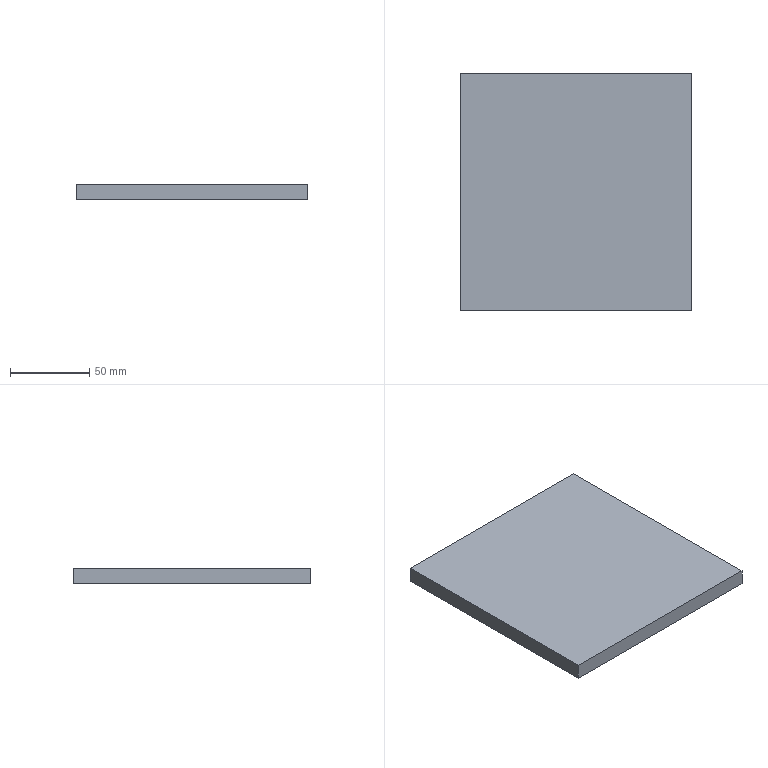Component | SolidWorks | THK-A1032DriveWheelSupportPlateReinforcementRib-1 | 1 solid | 6 faces | box 146 x 150 x 10 mm | volume 219000 mm3 | plane 6 | material Q235A
build123d program:
from build123d import *

# Parameters (mm, degrees)
SKETCH1_W           = 146
SKETCH1_H           = 150
BOSS_EXTRUDE1_DEPTH = 5


with BuildPart() as part:
    # Sketch1 → Boss-Extrude1 (new, symmetric)
    with BuildSketch(Plane.XY):
        Rectangle(SKETCH1_W, SKETCH1_H)
    extrude(amount=BOSS_EXTRUDE1_DEPTH, both=True)


solid = part.part

# Placed as in the assembly
solid = solid.moved(Location((0, 30, -20), (0, 0, 0)))
STEP:
#1=COLOUR_RGB('',0.7922,0.8196,0.9333);
#2=FILL_AREA_STYLE_COLOUR('',#1);
#3=FILL_AREA_STYLE('',(#2));
#4=SURFACE_STYLE_FILL_AREA(#3);
#5=SURFACE_SIDE_STYLE('',(#4));
#6=SURFACE_STYLE_USAGE(.BOTH.,#5);
#7=PRESENTATION_STYLE_ASSIGNMENT((#6));
#8=CARTESIAN_POINT('',(2.874,-1.772,-0.9843));
#9=VERTEX_POINT('',#8);
#10=CARTESIAN_POINT('',(2.874,4.134,-0.9843));
#11=VERTEX_POINT('',#10);
#12=CARTESIAN_POINT('',(2.874,-1.772,-0.9843));
#13=DIRECTION('',(0.,1.,0.));
#14=VECTOR('',#13,39.37);
#15=LINE('',#12,#14);
#16=EDGE_CURVE('',#9,#11,#15,.T.);
#17=ORIENTED_EDGE('',*,*,#16,.T.);
#18=CARTESIAN_POINT('',(2.874,4.134,-0.5906));
#19=VERTEX_POINT('',#18);
#20=CARTESIAN_POINT('',(2.874,4.134,-0.5906));
#21=DIRECTION('',(0.,0.,-1.));
#22=VECTOR('',#21,39.37);
#23=LINE('',#20,#22);
#24=EDGE_CURVE('',#19,#11,#23,.T.);
#25=ORIENTED_EDGE('',*,*,#24,.F.);
#26=CARTESIAN_POINT('',(2.874,-1.772,-0.5906));
#27=VERTEX_POINT('',#26);
#28=CARTESIAN_POINT('',(2.874,-1.772,-0.5906));
#29=DIRECTION('',(0.,1.,0.));
#30=VECTOR('',#29,39.37);
#31=LINE('',#28,#30);
#32=EDGE_CURVE('',#27,#19,#31,.T.);
#33=ORIENTED_EDGE('',*,*,#32,.F.);
#34=CARTESIAN_POINT('',(2.874,-1.772,-0.5906));
#35=DIRECTION('',(0.,0.,-1.));
#36=VECTOR('',#35,39.37);
#37=LINE('',#34,#36);
#38=EDGE_CURVE('',#27,#9,#37,.T.);
#39=ORIENTED_EDGE('',*,*,#38,.T.);
#40=EDGE_LOOP('',(#17,#25,#33,#39));
#41=FACE_OUTER_BOUND('',#40,.T.);
#42=CARTESIAN_POINT('',(2.874,-1.772,-0.5906));
#43=DIRECTION('',(-1.,0.,0.));
#44=DIRECTION('',(0.,0.,1.));
#45=AXIS2_PLACEMENT_3D('',#42,#43,#44);
#46=PLANE('',#45);
#47=ADVANCED_FACE('',(#41),#46,.F.);
#48=CARTESIAN_POINT('',(-2.874,4.134,-0.9843));
#49=VERTEX_POINT('',#48);
#50=CARTESIAN_POINT('',(-2.874,4.134,-0.9843));
#51=DIRECTION('',(-1.,0.,0.));
#52=VECTOR('',#51,39.37);
#53=LINE('',#50,#52);
#54=EDGE_CURVE('',#11,#49,#53,.T.);
#55=ORIENTED_EDGE('',*,*,#54,.T.);
#56=CARTESIAN_POINT('',(-2.874,4.134,-0.5906));
#57=VERTEX_POINT('',#56);
#58=CARTESIAN_POINT('',(-2.874,4.134,-0.5906));
#59=DIRECTION('',(0.,0.,-1.));
#60=VECTOR('',#59,39.37);
#61=LINE('',#58,#60);
#62=EDGE_CURVE('',#57,#49,#61,.T.);
#63=ORIENTED_EDGE('',*,*,#62,.F.);
#64=CARTESIAN_POINT('',(-2.874,4.134,-0.5906));
#65=DIRECTION('',(-1.,0.,0.));
#66=VECTOR('',#65,39.37);
#67=LINE('',#64,#66);
#68=EDGE_CURVE('',#19,#57,#67,.T.);
#69=ORIENTED_EDGE('',*,*,#68,.F.);
#70=ORIENTED_EDGE('',*,*,#24,.T.);
#71=EDGE_LOOP('',(#55,#63,#69,#70));
#72=FACE_OUTER_BOUND('',#71,.T.);
#73=CARTESIAN_POINT('',(-2.874,4.134,-0.5906));
#74=DIRECTION('',(0.,-1.,0.));
#75=DIRECTION('',(0.,0.,-1.));
#76=AXIS2_PLACEMENT_3D('',#73,#74,#75);
#77=PLANE('',#76);
#78=ADVANCED_FACE('',(#72),#77,.F.);
#79=CARTESIAN_POINT('',(-2.874,-1.772,-0.9843));
#80=VERTEX_POINT('',#79);
#81=CARTESIAN_POINT('',(-2.874,-1.772,-0.9843));
#82=DIRECTION('',(0.,-1.,0.));
#83=VECTOR('',#82,39.37);
#84=LINE('',#81,#83);
#85=EDGE_CURVE('',#49,#80,#84,.T.);
#86=ORIENTED_EDGE('',*,*,#85,.T.);
#87=CARTESIAN_POINT('',(-2.874,-1.772,-0.5906));
#88=VERTEX_POINT('',#87);
#89=CARTESIAN_POINT('',(-2.874,-1.772,-0.5906));
#90=DIRECTION('',(0.,0.,-1.));
#91=VECTOR('',#90,39.37);
#92=LINE('',#89,#91);
#93=EDGE_CURVE('',#88,#80,#92,.T.);
#94=ORIENTED_EDGE('',*,*,#93,.F.);
#95=CARTESIAN_POINT('',(-2.874,-1.772,-0.5906));
#96=DIRECTION('',(0.,-1.,0.));
#97=VECTOR('',#96,39.37);
#98=LINE('',#95,#97);
#99=EDGE_CURVE('',#57,#88,#98,.T.);
#100=ORIENTED_EDGE('',*,*,#99,.F.);
#101=ORIENTED_EDGE('',*,*,#62,.T.);
#102=EDGE_LOOP('',(#86,#94,#100,#101));
#103=FACE_OUTER_BOUND('',#102,.T.);
#104=CARTESIAN_POINT('',(-2.874,-1.772,-0.5906));
#105=DIRECTION('',(1.,0.,0.));
#106=DIRECTION('',(0.,0.,-1.));
#107=AXIS2_PLACEMENT_3D('',#104,#105,#106);
#108=PLANE('',#107);
#109=ADVANCED_FACE('',(#103),#108,.F.);
#110=CARTESIAN_POINT('',(-2.874,-1.772,-0.9843));
#111=DIRECTION('',(1.,0.,0.));
#112=VECTOR('',#111,39.37);
#113=LINE('',#110,#112);
#114=EDGE_CURVE('',#80,#9,#113,.T.);
#115=ORIENTED_EDGE('',*,*,#114,.T.);
#116=ORIENTED_EDGE('',*,*,#38,.F.);
#117=CARTESIAN_POINT('',(-2.874,-1.772,-0.5906));
#118=DIRECTION('',(1.,0.,0.));
#119=VECTOR('',#118,39.37);
#120=LINE('',#117,#119);
#121=EDGE_CURVE('',#88,#27,#120,.T.);
#122=ORIENTED_EDGE('',*,*,#121,.F.);
#123=ORIENTED_EDGE('',*,*,#93,.T.);
#124=EDGE_LOOP('',(#115,#116,#122,#123));
#125=FACE_OUTER_BOUND('',#124,.T.);
#126=CARTESIAN_POINT('',(-2.874,-1.772,-0.5906));
#127=DIRECTION('',(0.,1.,0.));
#128=DIRECTION('',(0.,0.,1.));
#129=AXIS2_PLACEMENT_3D('',#126,#127,#128);
#130=PLANE('',#129);
#131=ADVANCED_FACE('',(#125),#130,.F.);
#132=ORIENTED_EDGE('',*,*,#32,.T.);
#133=ORIENTED_EDGE('',*,*,#68,.T.);
#134=ORIENTED_EDGE('',*,*,#99,.T.);
#135=ORIENTED_EDGE('',*,*,#121,.T.);
#136=EDGE_LOOP('',(#132,#133,#134,#135));
#137=FACE_OUTER_BOUND('',#136,.T.);
#138=CARTESIAN_POINT('',(0.,1.181,-0.5906));
#139=DIRECTION('',(0.,0.,-1.));
#140=DIRECTION('',(-1.,0.,0.));
#141=AXIS2_PLACEMENT_3D('',#138,#139,#140);
#142=PLANE('',#141);
#143=ADVANCED_FACE('',(#137),#142,.F.);
#144=ORIENTED_EDGE('',*,*,#16,.F.);
#145=ORIENTED_EDGE('',*,*,#114,.F.);
#146=ORIENTED_EDGE('',*,*,#85,.F.);
#147=ORIENTED_EDGE('',*,*,#54,.F.);
#148=EDGE_LOOP('',(#144,#145,#146,#147));
#149=FACE_OUTER_BOUND('',#148,.T.);
#150=CARTESIAN_POINT('',(0.,1.181,-0.9843));
#151=DIRECTION('',(0.,0.,-1.));
#152=DIRECTION('',(-1.,0.,0.));
#153=AXIS2_PLACEMENT_3D('',#150,#151,#152);
#154=PLANE('',#153);
#155=ADVANCED_FACE('',(#149),#154,.T.);
#156=CLOSED_SHELL('',(#47,#78,#109,#131,#143,#155));
#157=MANIFOLD_SOLID_BREP('',#156);
#158=STYLED_ITEM('',(#7),#157);
#159=(LENGTH_UNIT()NAMED_UNIT(*)SI_UNIT($,.METRE.));
#160=LENGTH_MEASURE_WITH_UNIT(LENGTH_MEASURE(0.0254),#159);
#161=DIMENSIONAL_EXPONENTS(1.,0.,0.,0.,0.,0.,0.);
#162=(CONVERSION_BASED_UNIT('',#160)LENGTH_UNIT()NAMED_UNIT(#161));
#163=UNCERTAINTY_MEASURE_WITH_UNIT(LENGTH_MEASURE(0.00001),#162,'','');
#164=(NAMED_UNIT(*)PLANE_ANGLE_UNIT()SI_UNIT($,.RADIAN.));
#165=(NAMED_UNIT(*)SI_UNIT($,.STERADIAN.)SOLID_ANGLE_UNIT());
#166=(GEOMETRIC_REPRESENTATION_CONTEXT(3)GLOBAL_UNCERTAINTY_ASSIGNED_CONTEXT((#163))GLOBAL_UNIT_ASSIGNED_CONTEXT((#162,#164,#165))REPRESENTATION_CONTEXT('',''));
#167=MECHANICAL_DESIGN_GEOMETRIC_PRESENTATION_REPRESENTATION('',(#158),#166);
#168=CARTESIAN_POINT('',(0.,0.,0.));
#169=DIRECTION('',(0.,0.,1.));
#170=DIRECTION('',(1.,0.,0.));
#171=AXIS2_PLACEMENT_3D('',#168,#169,#170);
#172=(LENGTH_UNIT()NAMED_UNIT(*)SI_UNIT($,.METRE.));
#173=LENGTH_MEASURE_WITH_UNIT(LENGTH_MEASURE(0.0254),#172);
#174=DIMENSIONAL_EXPONENTS(1.,0.,0.,0.,0.,0.,0.);
#175=(CONVERSION_BASED_UNIT('',#173)LENGTH_UNIT()NAMED_UNIT(#174));
#176=UNCERTAINTY_MEASURE_WITH_UNIT(LENGTH_MEASURE(0.00001),#175,'','');
#177=(NAMED_UNIT(*)PLANE_ANGLE_UNIT()SI_UNIT($,.RADIAN.));
#178=(NAMED_UNIT(*)SI_UNIT($,.STERADIAN.)SOLID_ANGLE_UNIT());
#179=(GEOMETRIC_REPRESENTATION_CONTEXT(3)GLOBAL_UNCERTAINTY_ASSIGNED_CONTEXT((#176))GLOBAL_UNIT_ASSIGNED_CONTEXT((#175,#177,#178))REPRESENTATION_CONTEXT('',''));
#180=ADVANCED_BREP_SHAPE_REPRESENTATION('',(#157,#171),#179);
#181=PRESENTATION_LAYER_ASSIGNMENT('','',(#158));